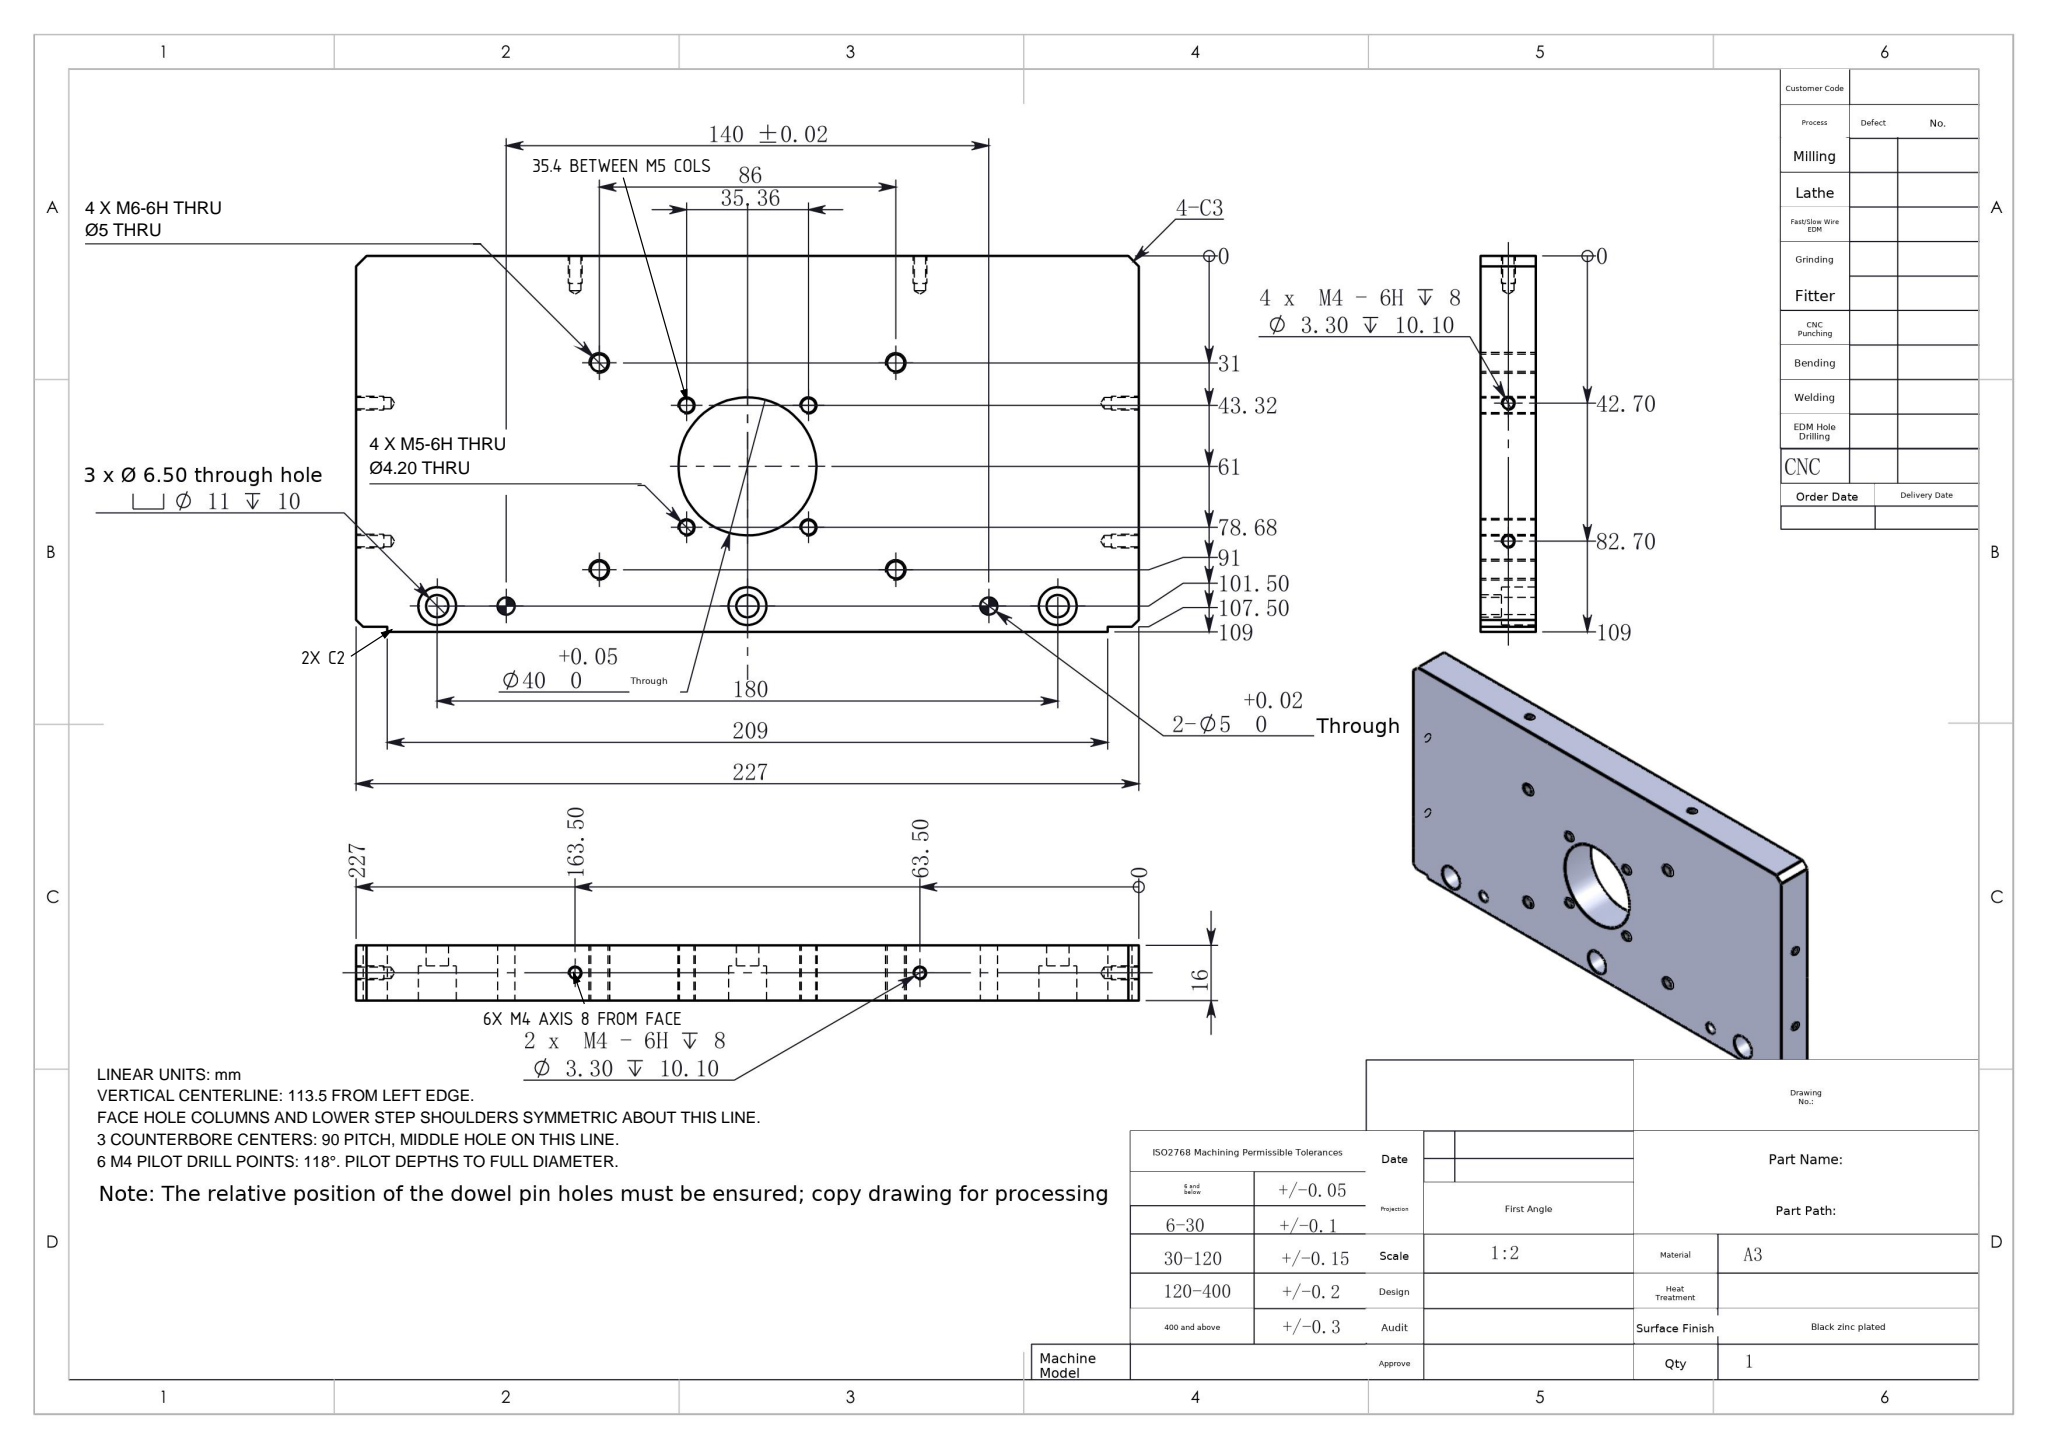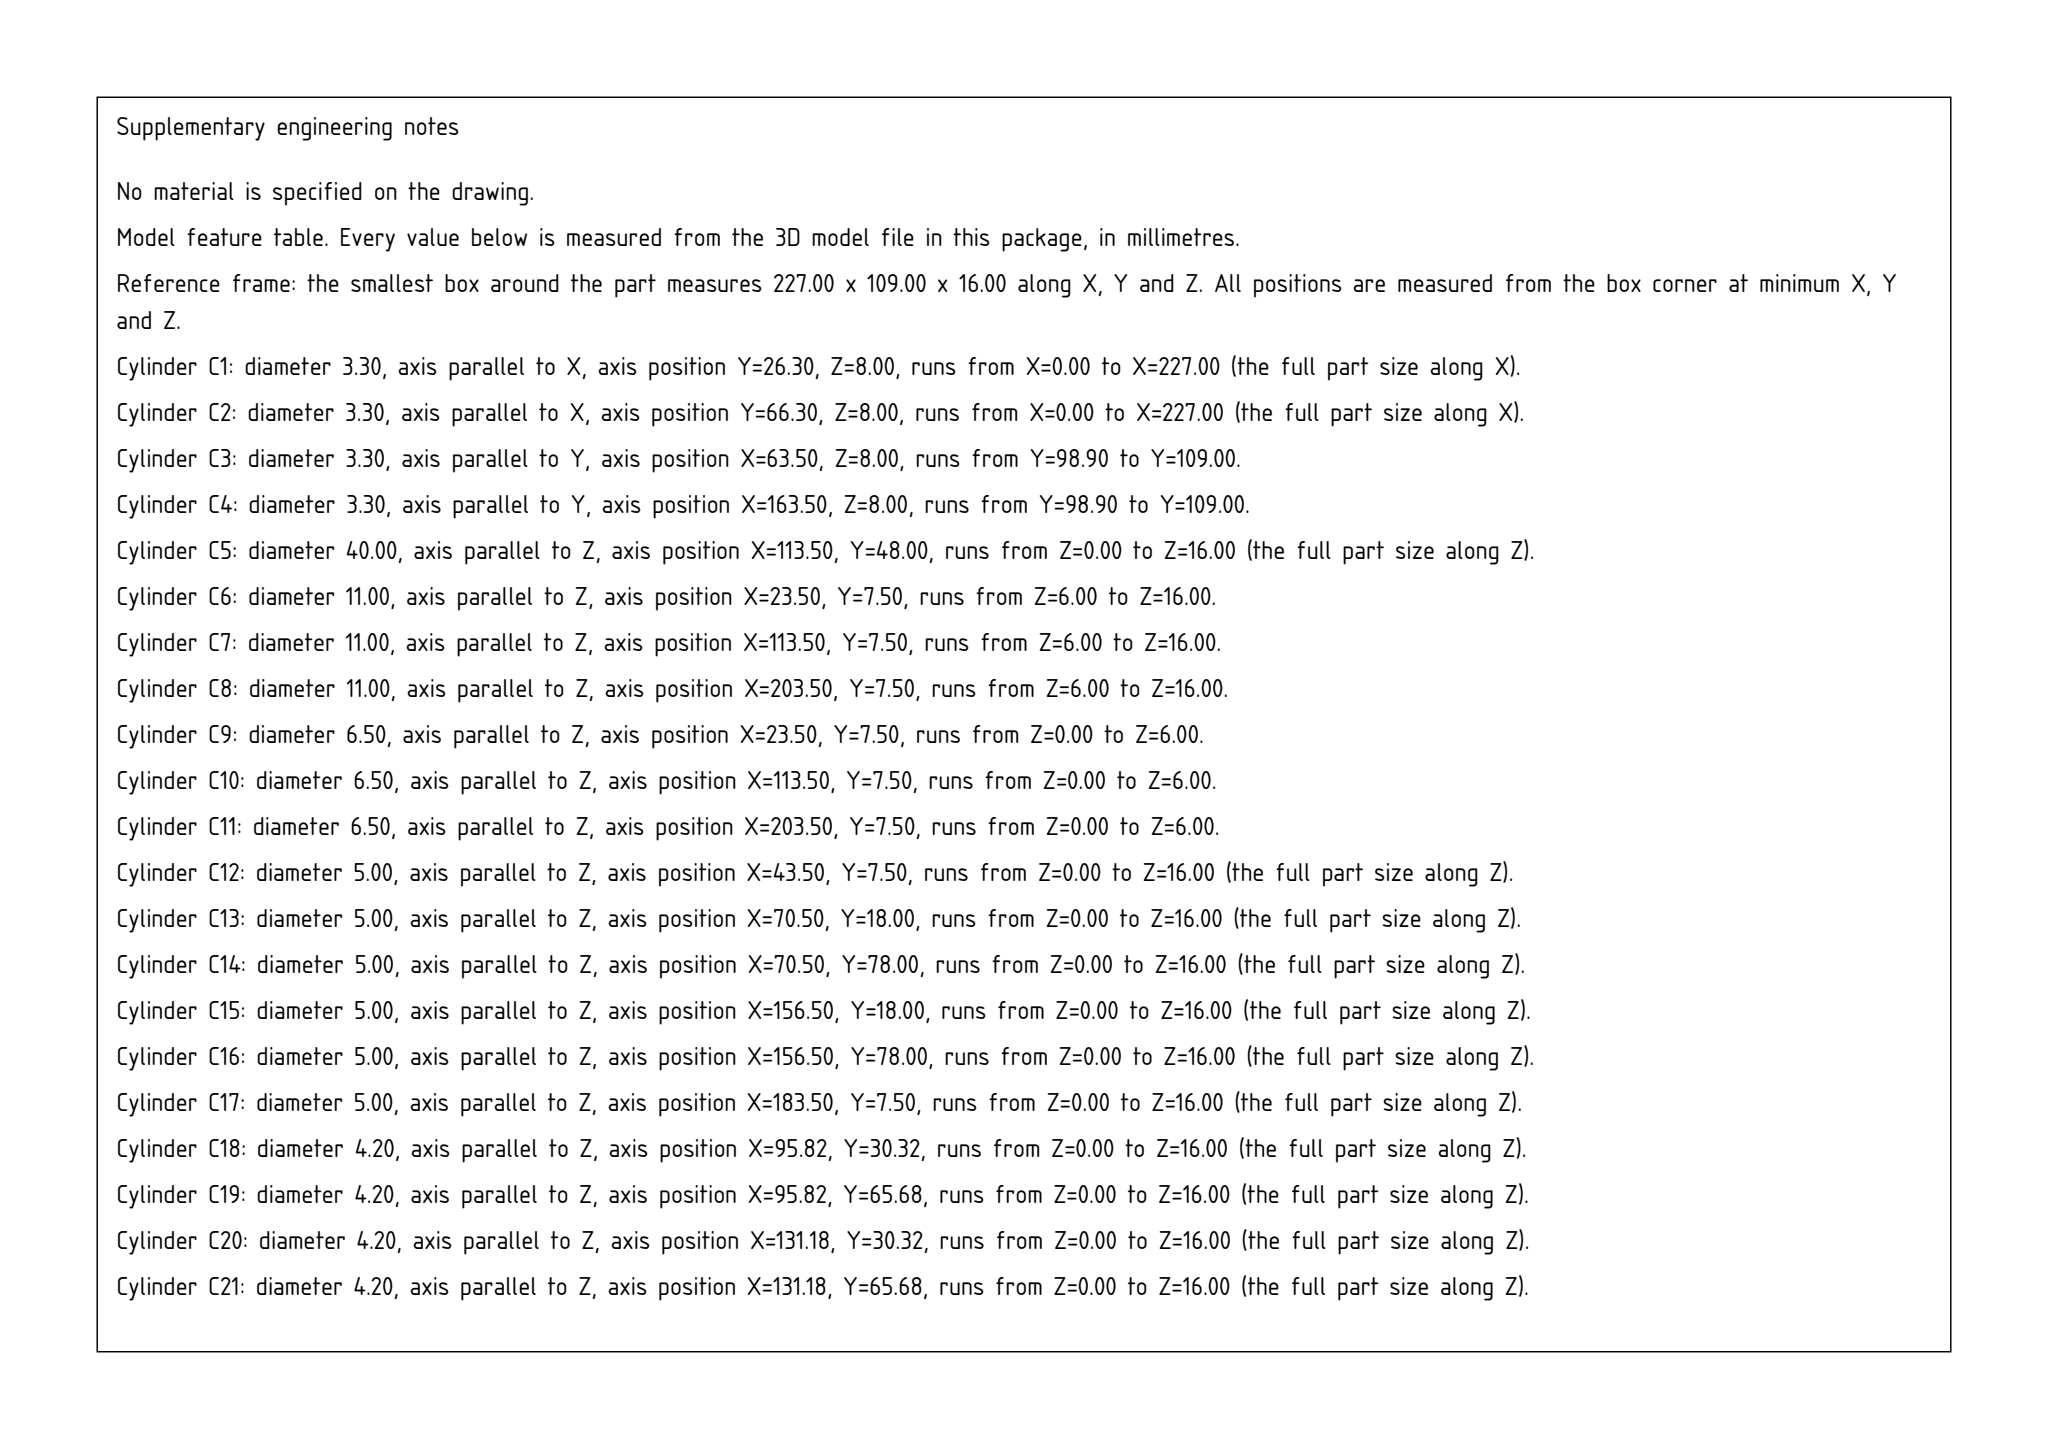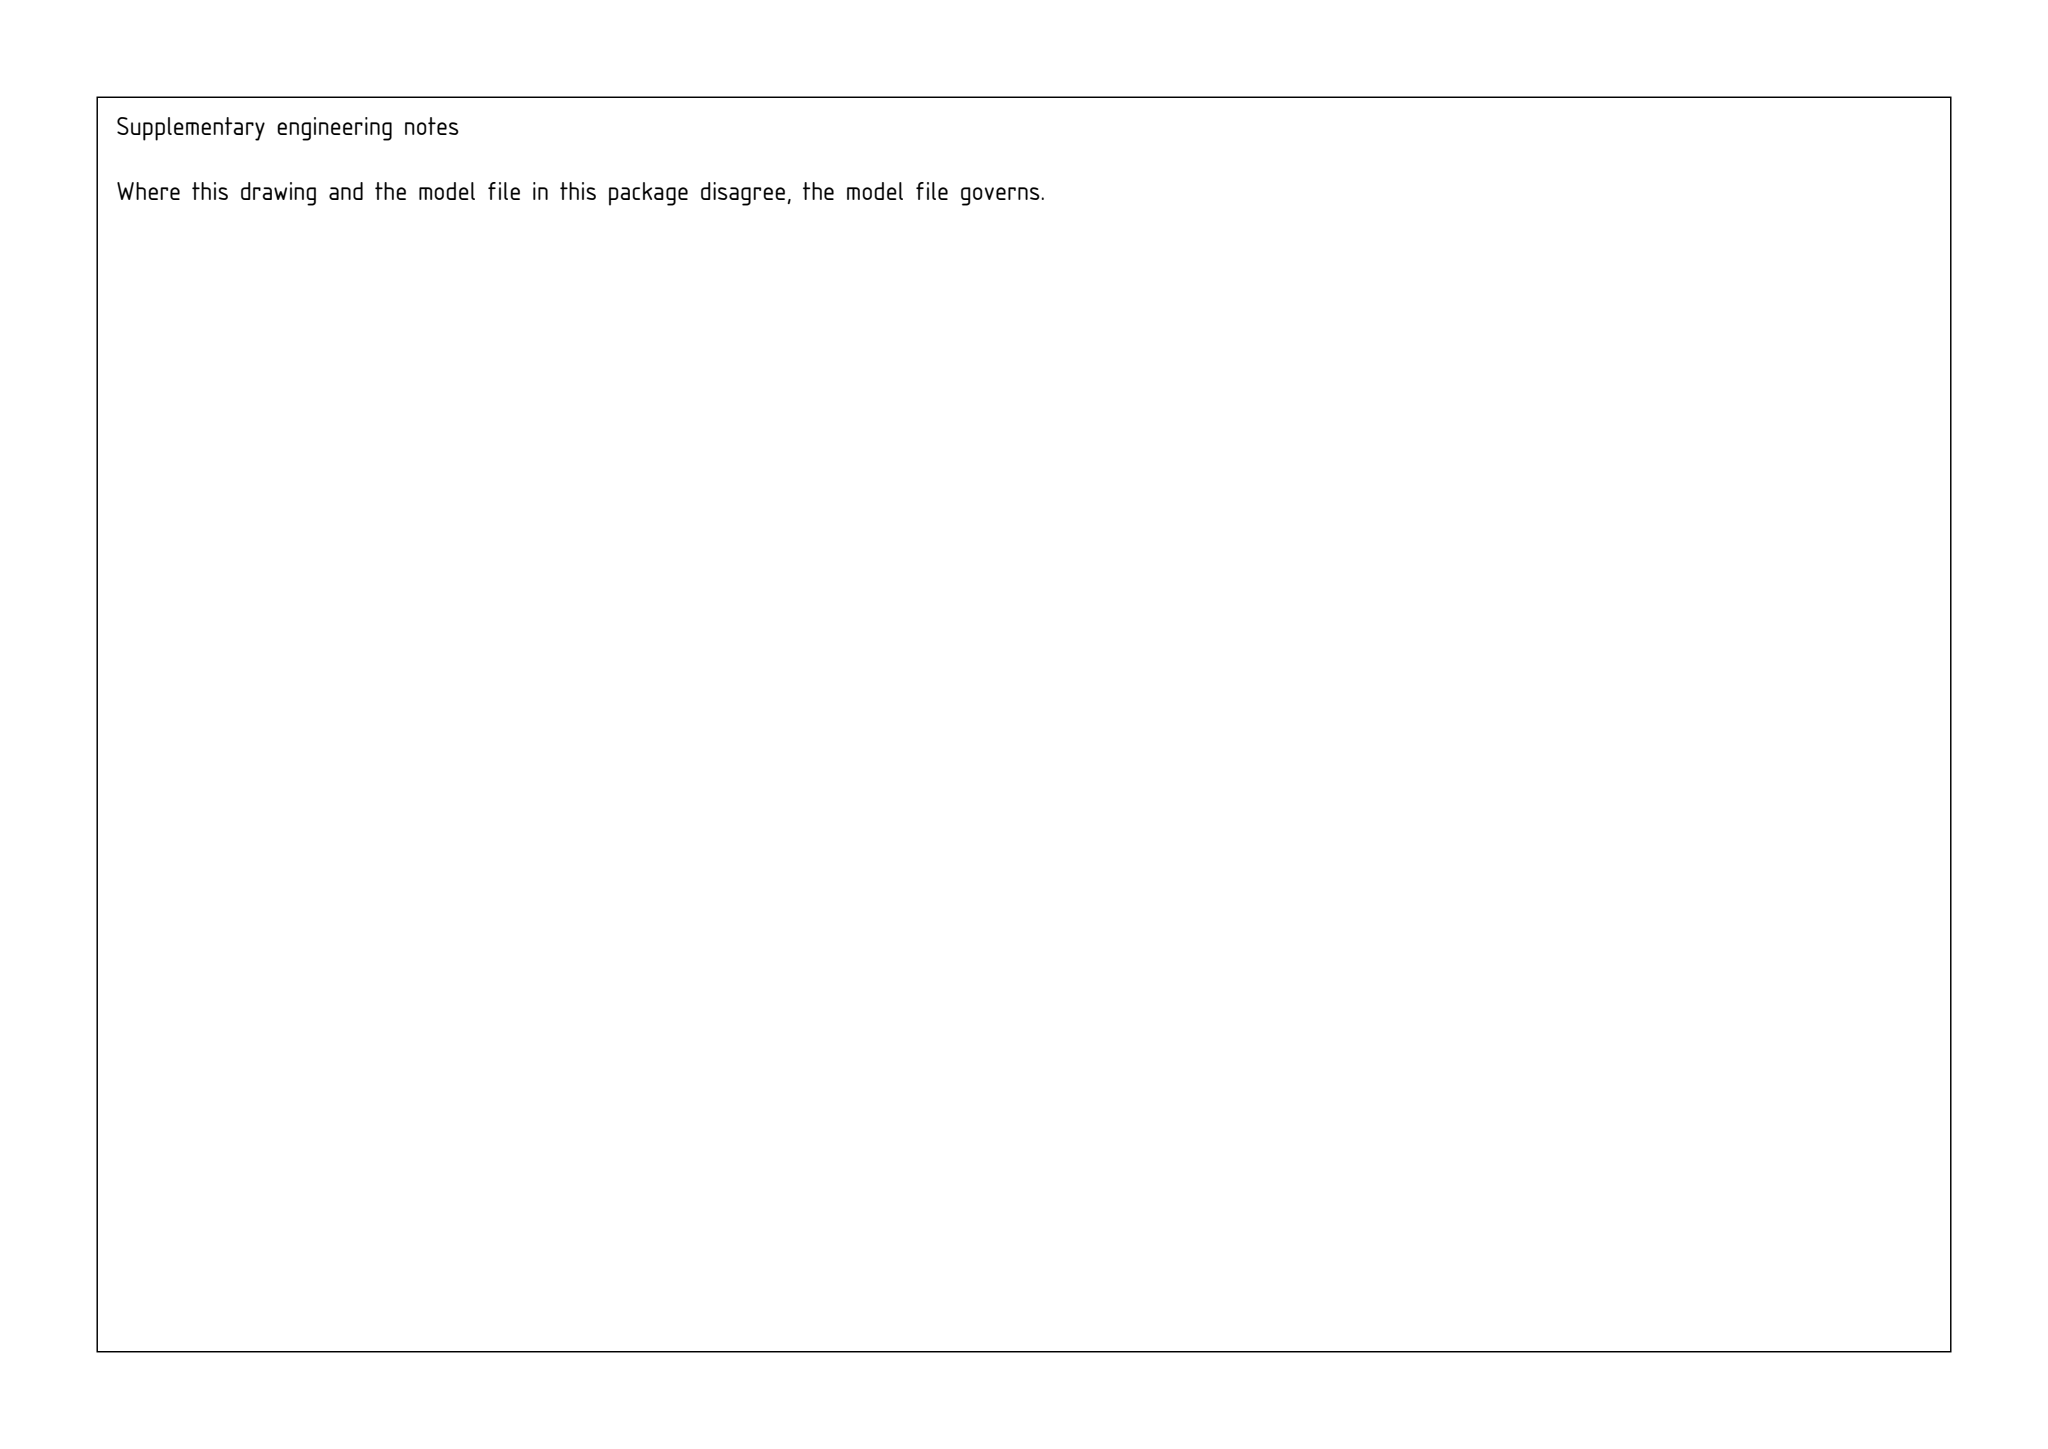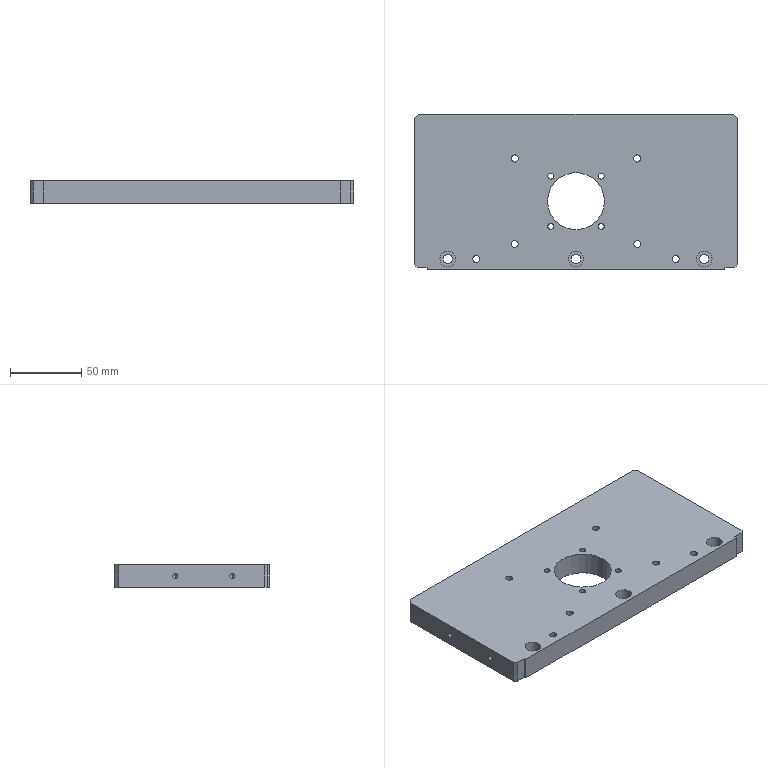Part | SolidWorks | mm | material A3 | 1 solid | 75 faces | box 227 x 109 x 16 mm | volume 368387 mm3 | cylinder 46 | plane 17 | cone 12 | commonest cylinder face diameters 5 x12 3.3 x12 4.2 x8 11 x6 6.5 x6 40 x2
Drawing notes:
2-C2 AT LOWER STEP-END CORNERS (4-C3 APPLIES TO OTHERS) | from the solid: Inclined 45 deg faces 2.0 x 2.0 x 16 at [0,1.5,0] and [225,1.5,0]; other two corners 3.0 x 3.0
6 x M4 TAPPED HOLES: AXES AT 8 FROM FACE (MID OF 16 THK) | from the solid: Ø3.3 holes along x at [y26.3,z8.0] & [y66.3,z8.0]; along y at [x163.5,z8.0] & [x63.5,z8.0]; plate z 0-16
"35, 36" = 35.4 BETWEEN M5 COLS (17.7 EA SIDE OF CL 113.5) | from the solid: Ø4.2 holes at x=95.8 and x=131.2; 131.2-95.8=35.4, symmetric about x=113.5
build123d program:
from build123d import *

# Parameters (mm, degrees)
SKETCH4_W                                          = 227
SKETCH4_H                                          = 109
SKETCH4_R                                          = 20
SKETCH4_R_2                                        = 2.5
BOSS_EXTRUDE1_DEPTH                                = 16
CHAMFER1_SIZE                                      = 3
HOLE_SIZE_ACCORDING_TO_TYPE_1_OF_HEXAG_D           = 6.5
HOLE_SIZE_ACCORDING_TO_TYPE_1_OF_HEXAG_CBORE_D     = 11
HOLE_SIZE_ACCORDING_TO_TYPE_1_OF_HEXAG_CBORE_DEPTH = 10
M4_TAPPED_HOLE1_AT_2_COUNT                         = 2
M4_TAPPED_HOLE1_AT_2_PITCH                         = 40
M4_TAPPED_HOLE3_D                                  = 3.3
M4_TAPPED_HOLE3_DEPTH                              = 10.1
M4_TAPPED_HOLE3_TIP                                = 0.9914
M4_TAPPED_HOLE2_D                                  = 3.3
M4_TAPPED_HOLE2_DEPTH                              = 10.1
M4_TAPPED_HOLE2_TIP                                = 0.9914
SKETCH15_W                                         = 9
SKETCH15_H                                         = 1.5
CUT_EXTRUDE2_DEPTH                                 = 65
CHAMFER2_SIZE                                      = 2
M5_TAPPED_HOLE1_D                                  = 4.2
M6_TAPPED_HOLE1_D                                  = 5


with BuildPart() as part:
    # Sketch4 → Boss-Extrude1 (new body)
    with BuildSketch(Plane.XY):
        Rectangle(SKETCH4_W, SKETCH4_H)
        with Locations((0, -6.5)):
            Circle(SKETCH4_R, mode=Mode.SUBTRACT)
        with Locations((-70, -47)):
            Circle(SKETCH4_R_2, mode=Mode.SUBTRACT)
        with Locations(Location((70, -47, 0), (0, 0, 180))):
            Circle(SKETCH4_R_2, mode=Mode.SUBTRACT)
    extrude(amount=BOSS_EXTRUDE1_DEPTH)

    # Chamfer1
    chamfer1_edges = [part.edges().sort_by_distance(p)[0] for p in [
        (-113.5, 54.5, 8),
        (113.5, 54.5, 8),
    ]]
    chamfer(chamfer1_edges, length=CHAMFER1_SIZE)

    # Hole Size _according to_ Type 1 of Hexag (through all)
    with Locations(Plane.XY.offset(16)):
        with Locations((90, -47), (-90, -47), (0, -47)):
            CounterBoreHole(HOLE_SIZE_ACCORDING_TO_TYPE_1_OF_HEXAG_D / 2, HOLE_SIZE_ACCORDING_TO_TYPE_1_OF_HEXAG_CBORE_D / 2, HOLE_SIZE_ACCORDING_TO_TYPE_1_OF_HEXAG_CBORE_DEPTH)

    # Sketch12 → M4 Tapped Hole1 (revolve, cut)
    with BuildSketch(Plane(origin=(113.5, -28.2, 8), x_dir=(0, 0, -1), z_dir=(0, 1, 0))):
        Polygon((0, 0), (0, 11.091), (1.65, 10.1), (1.65, 0), align=None)
    m4_tapped_hole1 = revolve(axis=Axis((119.85, -28.2, 8), (-1, 0, 0)), mode=Mode.SUBTRACT)

    # M4 Tapped Hole1 at 2: M4 Tapped Hole1 ×2
    with Locations(*[(0, i * M4_TAPPED_HOLE1_AT_2_PITCH, 0) for i in range(1, M4_TAPPED_HOLE1_AT_2_COUNT)]):
        add(m4_tapped_hole1, mode=Mode.SUBTRACT)

    # M4 Tapped Hole3
    with Locations(Plane(origin=(0, 54.5, 0), x_dir=(1, 0, 0), z_dir=(0, 1, 0))):
        with Locations((-50, -8), (50, -8)):
            Hole(M4_TAPPED_HOLE3_D / 2, depth=M4_TAPPED_HOLE3_DEPTH)
            with Locations((0, 0, -(M4_TAPPED_HOLE3_DEPTH + M4_TAPPED_HOLE3_TIP / 2))):  # 118° drill point
                Cone(0, M4_TAPPED_HOLE3_D / 2, M4_TAPPED_HOLE3_TIP, mode=Mode.SUBTRACT)

    # M4 Tapped Hole2
    with Locations(Plane(origin=(0, 54.5, 0), x_dir=(1, 0, 0), z_dir=(0, 1, 0))):
        with Locations((-50, -8), (50, -8)):
            Hole(M4_TAPPED_HOLE2_D / 2, depth=M4_TAPPED_HOLE2_DEPTH)
            with Locations((0, 0, -(M4_TAPPED_HOLE2_DEPTH + M4_TAPPED_HOLE2_TIP / 2))):  # 118° drill point
                Cone(0, M4_TAPPED_HOLE2_D / 2, M4_TAPPED_HOLE2_TIP, mode=Mode.SUBTRACT)

    # Sketch15 → Cut-Extrude2 (cut)
    with BuildSketch(Plane.XY.offset(16)):
        with Locations((-109, -53.75)):
            Rectangle(SKETCH15_W, SKETCH15_H)
        with Locations((109, -53.75)):
            Rectangle(SKETCH15_W, SKETCH15_H)
    extrude(amount=-CUT_EXTRUDE2_DEPTH, mode=Mode.SUBTRACT)

    # Chamfer2
    chamfer2_edges = [part.edges().sort_by_distance(p)[0] for p in [
        (113.5, -53, 8),
        (-113.5, -53, 8),
    ]]
    chamfer(chamfer2_edges, length=CHAMFER2_SIZE)

    # M5 Tapped Hole1 (through all)
    with Locations(Plane.XY.offset(16)):
        with Locations((-17.678, 11.178), (17.678, 11.178), (17.678, -24.178), (-17.678, -24.178)):
            Hole(M5_TAPPED_HOLE1_D / 2)

    # Mirror1: M4 Tapped Hole1 across plane
    add(m4_tapped_hole1.mirror(Plane(origin=(0, 0, 0), x_dir=(0, 0, 1), z_dir=(1, 0, 0))), mode=Mode.SUBTRACT)

    # Mirror1 copy 1 sketch → Mirror1 copy 1 (revolve, cut)
    with BuildSketch(Plane(origin=(-113.5, 11.8, 8), x_dir=(0, 0, -1), z_dir=(0, 1, 0))):
        Polygon((0, 0), (0, -11.091), (1.65, -10.1), (1.65, 0), align=None)
    revolve(axis=Axis((-119.85, 11.8, 8), (-1, 0, 0)), mode=Mode.SUBTRACT)

    # M6 Tapped Hole1 (through all)
    with Locations(Plane.XY.offset(16)):
        with Locations((-43, 23.5), (43, 23.5), (43, -36.5), (-43, -36.5)):
            Hole(M6_TAPPED_HOLE1_D / 2)


solid = part.part